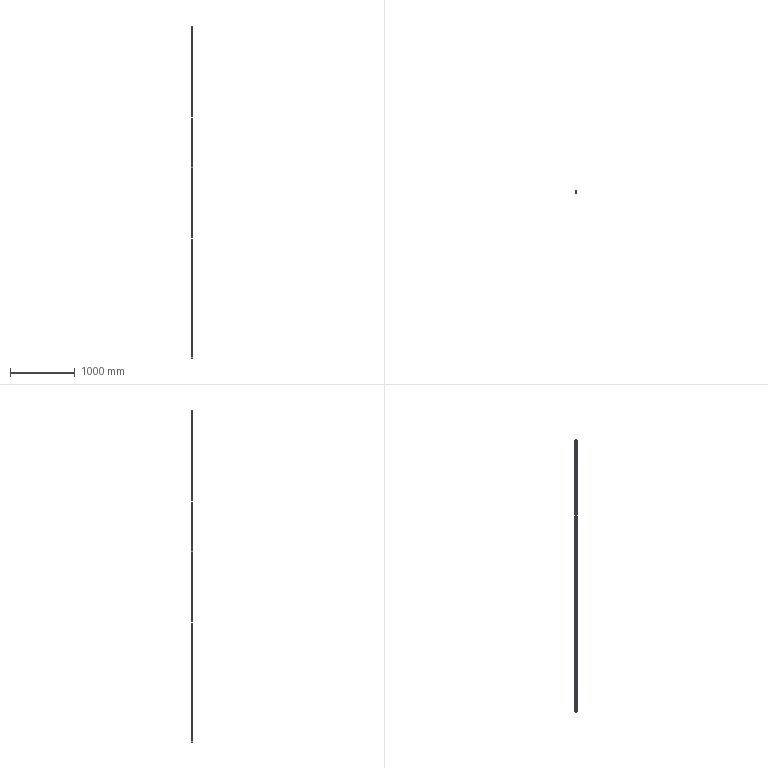Component | SolidWorks | MirrorRailing-2-3_Mirror30X30X3-3720-30-1 | 3 solids | 54 faces | volume 1522164 mm3 | plane 30 | cylinder 24 | commonest cylinder face diameters 12 x12 6 x12